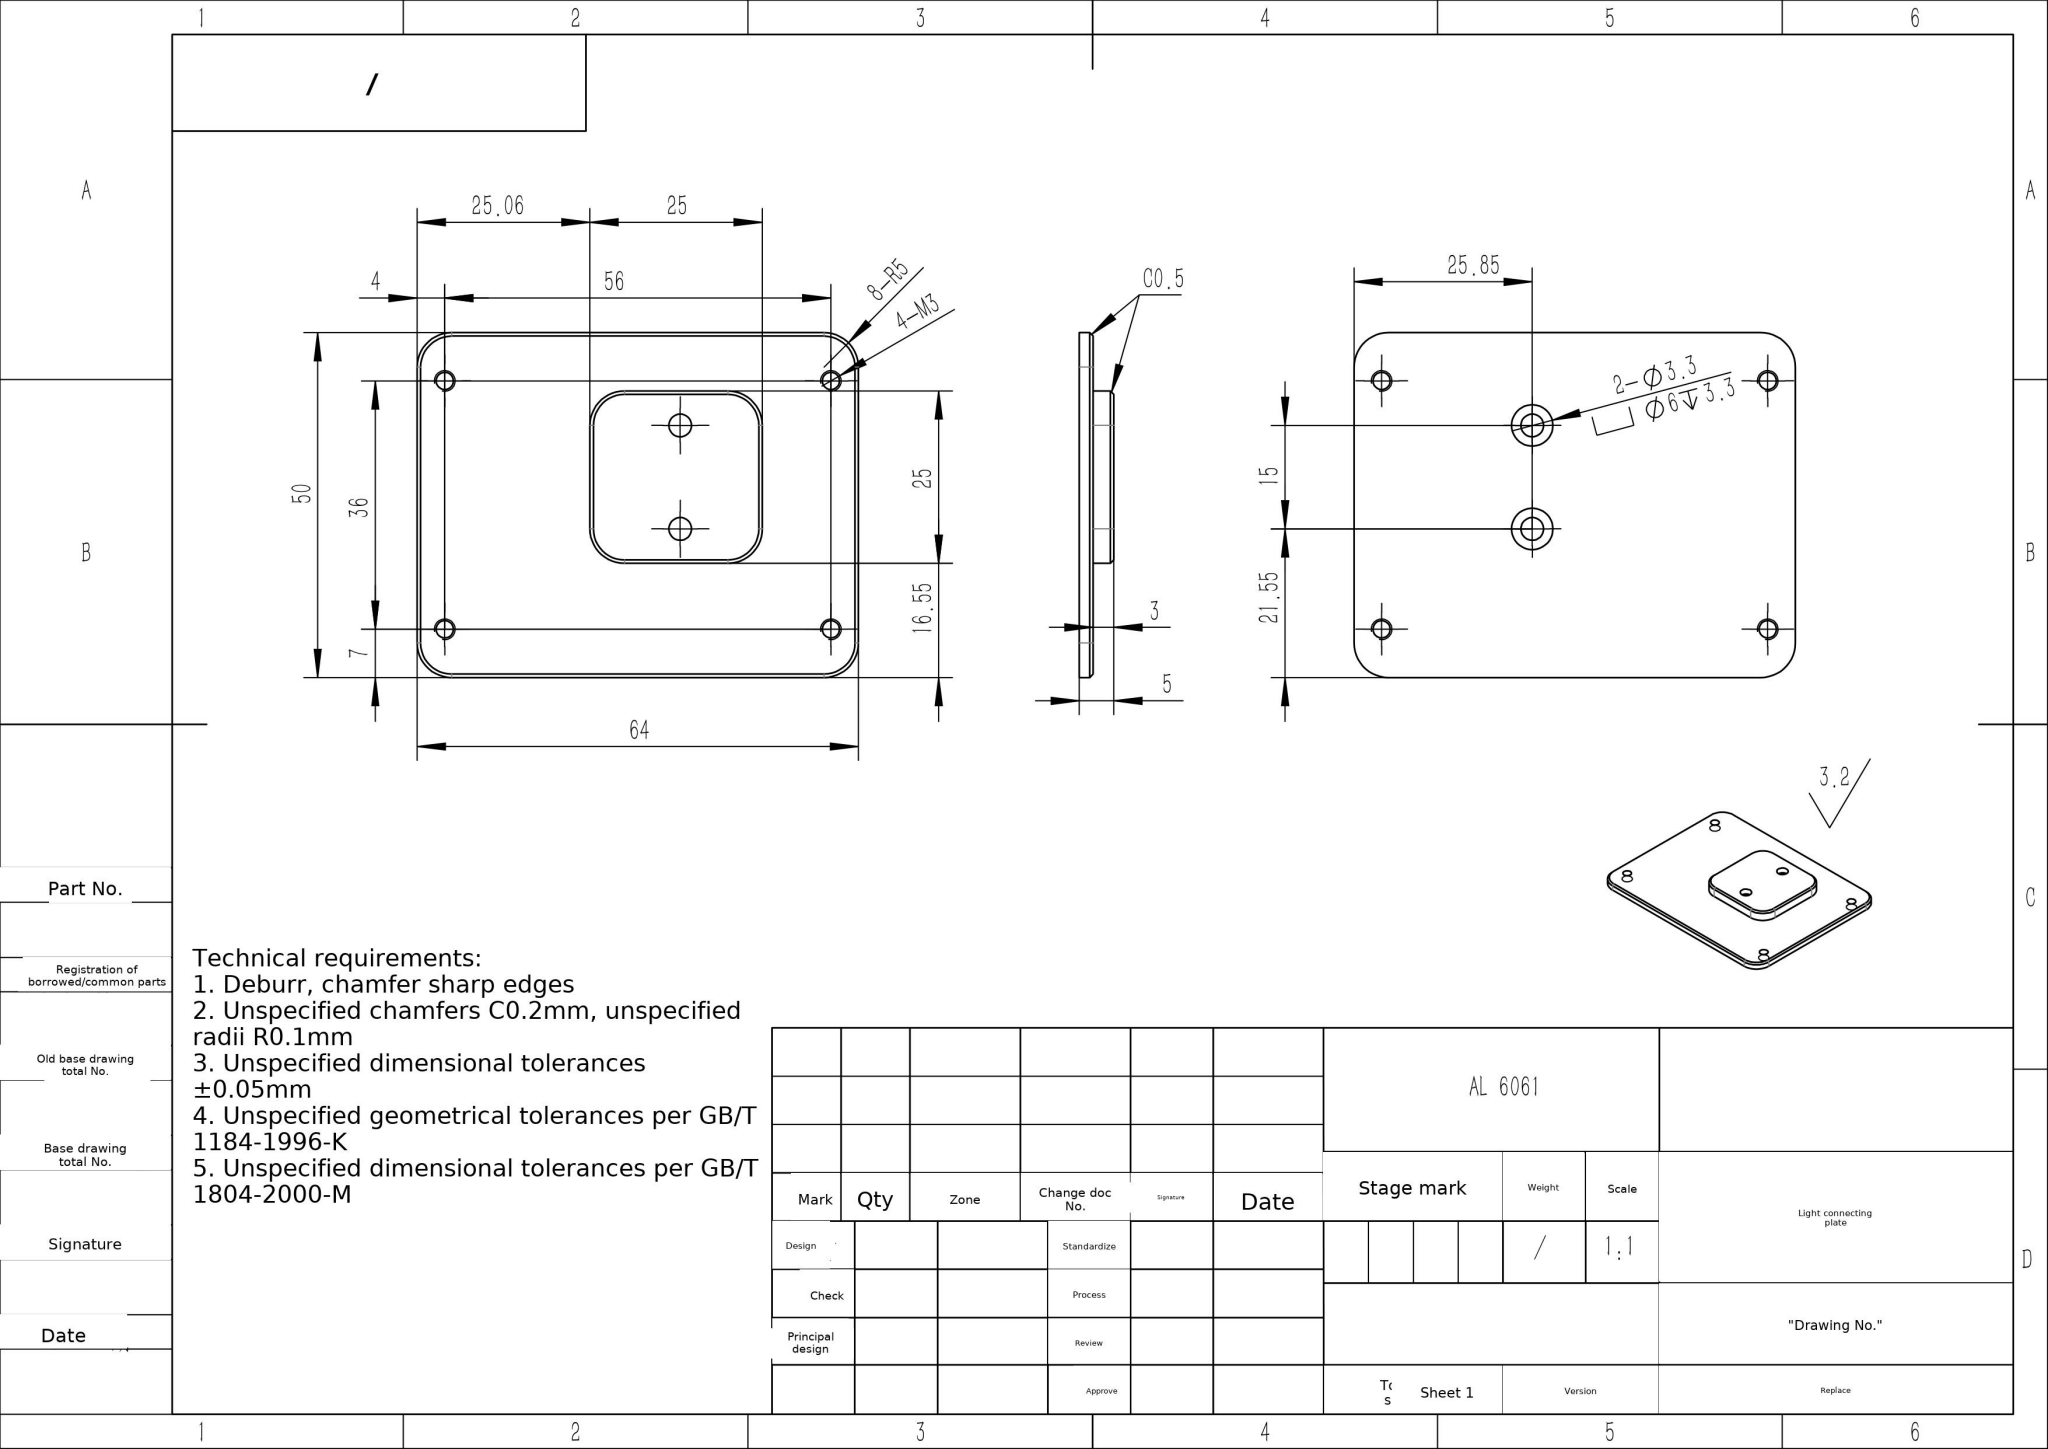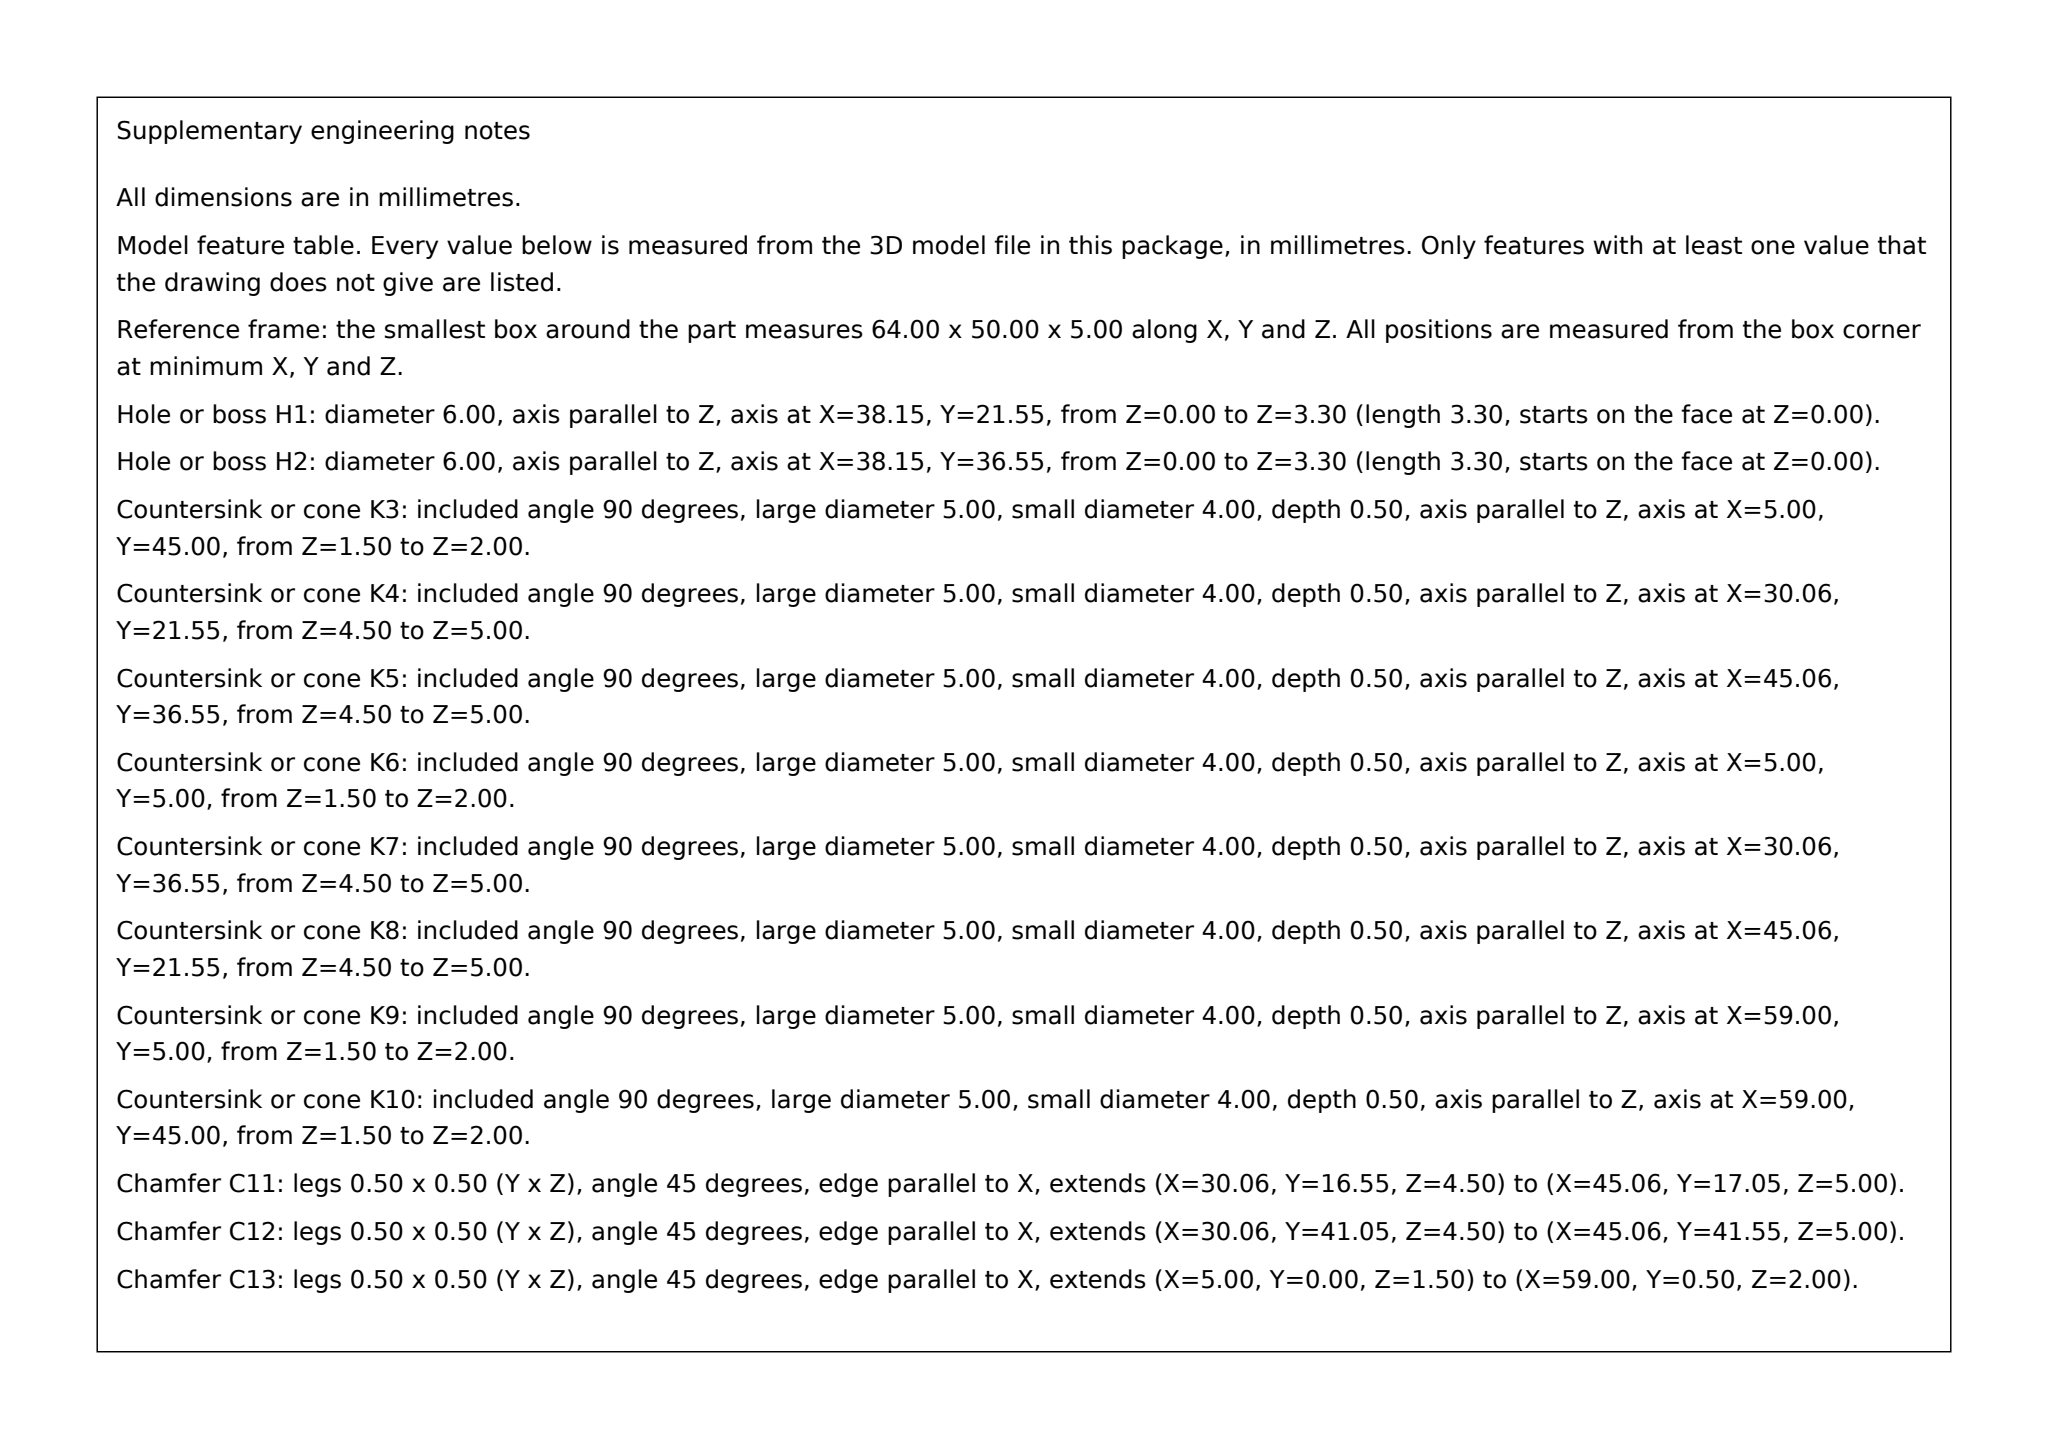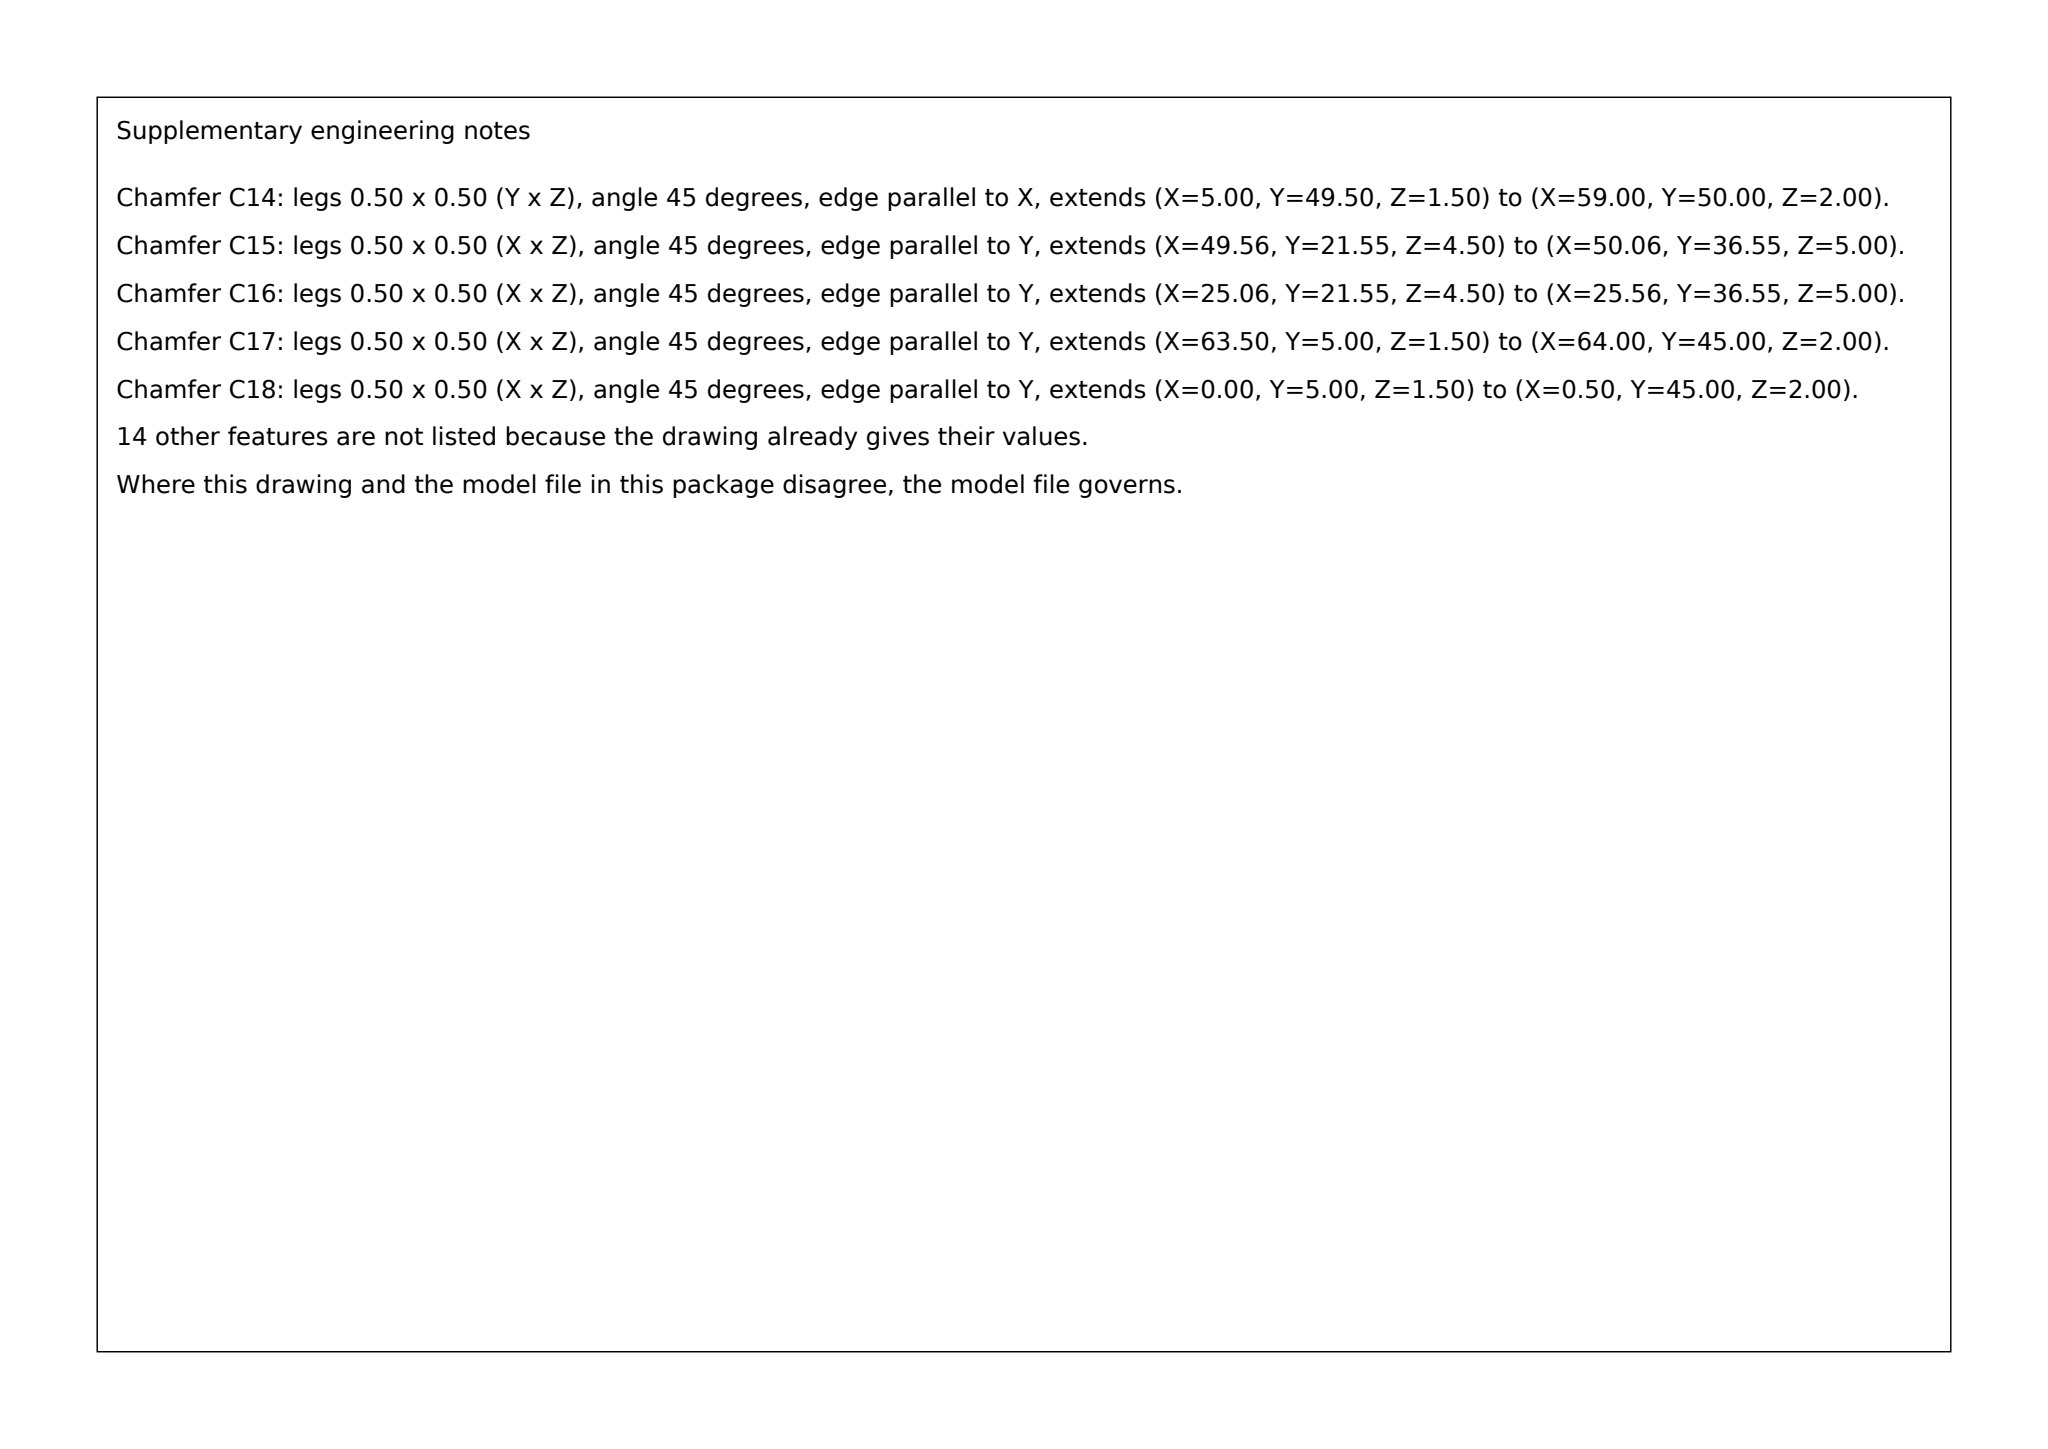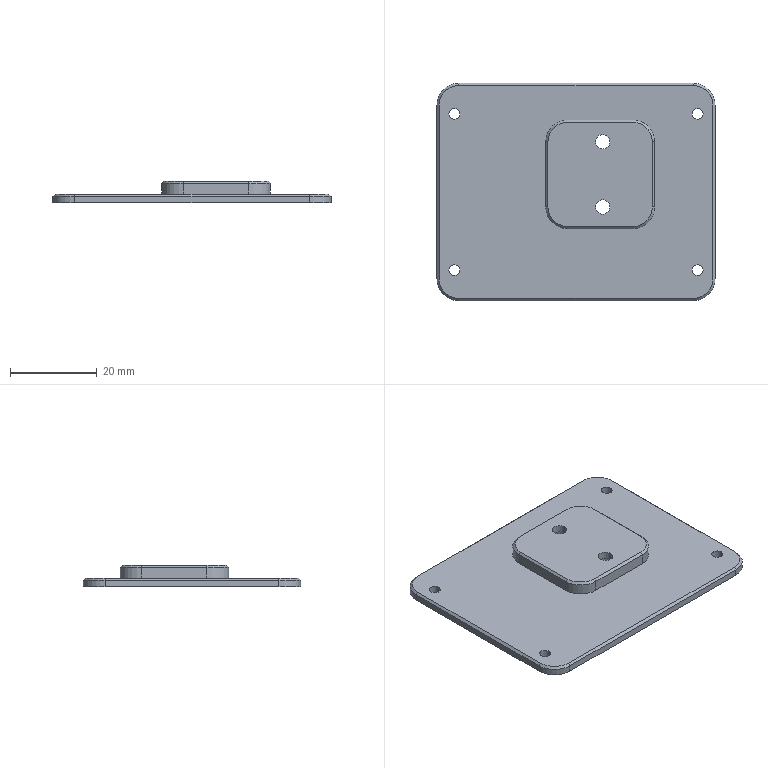Part | SolidWorks | mm | material AL 6061 | 1 solid | 53 faces | box 64 x 50 x 5 mm | volume 7874 mm3 | cylinder 24 | plane 21 | cone 8 | commonest cylinder face diameters 2.5 x8 10 x8 6 x4 3.3 x4